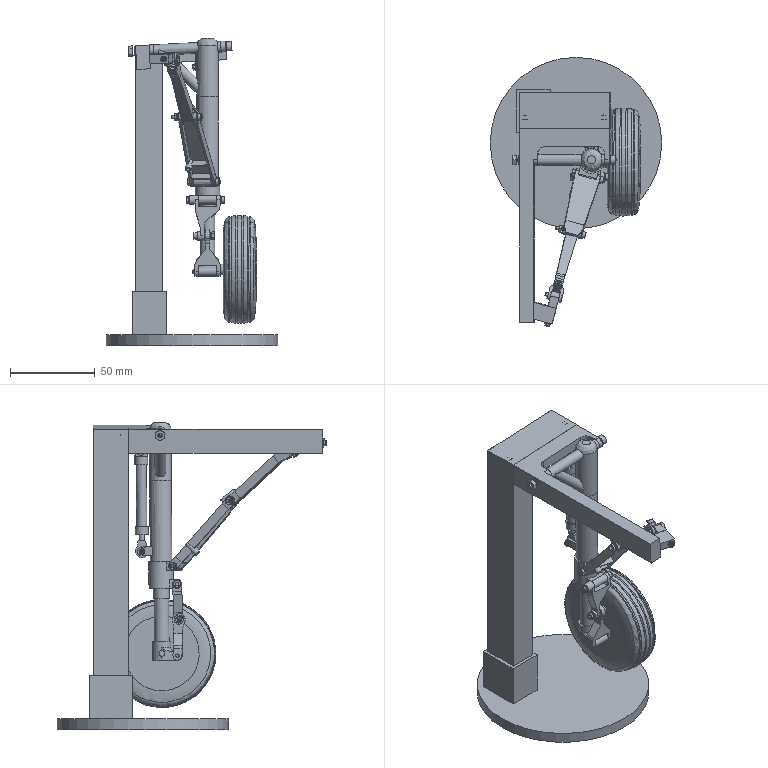Assembly | NX | mm | 58 component files | 58 solids | 973 faces | box 101 x 158.93 x 181.11 mm | volume 209079 mm3 | plane 512 | cone 218 | cylinder 196 | torus 33 | spline 10 | sphere 4 | commonest cylinder face diameters 2 x26 5.292 x14 6.35 x14 12.7 x9 3.3 x9 3.35 x8 2.35 x8 1.587 x6
Bill of materials:
GB93-87,2 | 8 |  | Single Coil Spring Lock Washer, Normal Type, GB 93-87,2
GB-T848-2002,M2 | 6 |  | Thin, flat ring (annular disc) with a single concentric through-hole; looks like a plain flat washer.
unnamed part 1 | 1 |  | Y-shaped or triangular plate bracket. Two widely spaced lugs with holes form a forked top, and the body tapers down to a single lug with a hole at the bottom.
unnamed part 2 | 1 |  | Long, slightly tapered channel or frame arm. Twin parallel side plates are joined by cross webs, and each end has a forked pair of lugs with holes. A small cylindrical boss sticks out from one side.
unnamed part 3 | 1 |  | Inverted-L (gamma-shaped) bar of rectangular cross-section: a long vertical leg with a short horizontal arm at the top. Small holes are visible near the corner and at the arm end.
unnamed part 4 | 1 |  | Wheel with tyre: a rounded toroidal tread with several circumferential grooves around a recessed central hub disc that has a small central bore.
GB-T70.1-2000,M2x20 | 1 |  | Hexagon Socket Head Cap Screw, GB-T 70.1-2000,M2x20
unnamed part 5 | 2 |  | Sphere truncated by two parallel flat faces and pierced by a central through-bore along the axis normal to those faces. It resembles a ball-joint ball or bead.
unnamed part 6 | 1 |  | Thin circular disc base with a hollow square tube standing upright on it, offset from the disc centre.
unnamed part 7 | 1 |  | Long rectangular bar with a hook- or C-shaped end. The end returns into a bracket with holed lugs and a slot, and a small angled block with a hole sits near the opposite end.
unnamed part 8 | 1 |  | Clevis or fork bracket: two parallel lugs with coaxial holes rising from a rounded base. The base has a larger cross hole and a U-shaped slot between the lugs.
unnamed part 9 | 1 |  | Hollow cylindrical tube with a pair of small parallel tabs near one end. The tabs have holes and form a small fork on the tube side.
unnamed part 10 | 1 |  | Tubular frame node: a vertical round post with a domed or ball-shaped top. A horizontal round bar passes through the top, and a diagonal brace runs from the bar to the post. A small bossed hole sits on the dome.
GB-T6170_F-2000,M3x0.5 | 1 |  | Hexagonal nut-like body with a central round bore and chamfered corners on both faces.
GB-T119.1-2000,2x10 | 1 |  | Parallel Pin, GB-T 119.1-2000,2x10
GB-T6170_F-2000,M1.6x0.35 | 2 |  | Hexagonal nut-like body with a central round bore and chamfered corners on both faces.
GB93-87,3 | 2 |  | Single Coil Spring Lock Washer, Normal Type, GB 93-87,3
unnamed part 11 | 1 |  | Cylindrical sleeve with a large axial through-bore and two flat lugs with rounded ends sticking out sideways. The lugs sit at different heights and point in slightly different directions, and each has a small through-hole.
unnamed part 12 | 1 |  | Tee-shaped body: a vertical cylindrical boss with an open, hollow top bore, a flat rounded-end lug with a small through-hole, and a short side boss with a larger through-hole. The side boss axis runs at right angles to the vertical boss. The joins between features are smoothly filleted.
unnamed part 13 | 1 |  | Flat Y-shaped forked lever. One end is a single rounded eye with a larger hole. A narrow stem widens into a two-prong fork at the other end, and each prong ends in a rounded tip with a small hole.
unnamed part 14 | 1 |  | Long, straight, thin-walled round tube with plain square-cut ends.
unnamed part 15 | 1 |  | Rectangular block with one end rounded into a semicircle. One through-hole runs across the rounded end, square to the large side faces. A second hole enters the flat square end face.
GB-T119.1-2000,2x16 | 1 |  | Parallel Pin, GB-T 119.1-2000,2x16
unnamed part 16 | 1 |  | Long, straight, thin-walled round tube with plain square-cut ends.
GB-T70.1-2000,M3x30 | 1 |  | Hexagon Socket Head Cap Screw, GB-T 70.1-2000,M3x30
unnamed part 17 | 1 |  | Slender solid round rod with a flat eyelet lug at one end. The lug has a through-hole whose axis is square to the rod axis.
GB-T6170_F-2000,M2x0.4 | 5 |  | Hexagonal prism with a round central through-hole. The corners are chamfered on both faces, which gives curved arcs on the side flats. It looks like a hex nut.
GB-T70.1-2000,M1.6x10 | 3 |  | Hexagon Socket Head Cap Screw, GB-T 70.1-2000,M1.6x10
unnamed part 18 | 1 |  | Slender cylindrical body with a larger-diameter collar at each end. A flat tab with a small cross-hole sticks out from one end collar.
GB-T70.1-2000,M3x5 | 3 |  | Hexagon Socket Head Cap Screw, GB-T 70.1-2000,M3x5
GB-T70.1-2000,M2x16 | 2 |  | Hexagon Socket Head Cap Screw, GB-T 70.1-2000,M2x16
GB-T70.1-2000,M2x10 | 2 |  | Hexagon Socket Head Cap Screw, GB-T 70.1-2000,M2x10
unnamed part 19 | 1 |  | Long, flat, slightly tapered arm. One end is a two-prong fork with a small hole in each prong tip. The other end has a rounded boss with a hole and a stepped, angled tab.
Mates:
1. fix | base 1 component
2. touch align | support_rod 1 face | base 1 face
3. center | support_rod 1 face | support_rod 1 face | base 1 face | base 1 face
4. center | support_rod 1 face | support_rod 1 face | base 1 face | base 1 face
5. concentric | main_frame 1 edge | support_rod 1 edge
6. concentric | bearing_housing 1 edge | main_frame 1 edge
7. concentric | casing 1 edge | bearing_housing 1 edge
8. parallel | main_frame 1 face | support_rod 1 face
9. concentric | connecting_block 1 edge | casing 1 edge
10. concentric | block 1 edge | main_frame 1 edge
11. center | universal_joint_1 1 face | universal_joint_1 1 face | block 1 face | block 1 face
12. touch align | universal_joint_1 1 face | block 1 face
13. center | connecting_rod_2 1 face | connecting_rod_2 1 face | universal_joint_1 1 face | universal_joint_1 1 face
14. touch align | connecting_rod_2 1 face | universal_joint_1 1 face
15. center | connecting_rod 1 face | connecting_rod 1 face | connecting_rod_2 1 face | connecting_rod_2 1 face
16. touch align | connecting_rod 1 face | connecting_rod_2 1 face
17. touch align | connecting_rod 1 face | connecting_block 1 face
18. center | connecting_rod 1 face | connecting_rod 1 face | connecting_block 1 face | connecting_block 1 face
19. touch align | rotating_rod_2 1 face | connecting_block 1 face
20. center | rotating_rod_2 1 face | rotating_rod_2 1 face | connecting_block 1 face | connecting_block 1 face
21. touch align | tube_2 1 face | casing 1 face
22. touch align | tube_1 1 face | tube_2 1 face
23. distance | tube_2 1 face | connecting_block 1 face
24. touch align | support 1 face | tube_1 1 face
25. fit | ball_1 2 face | rotating_rod 1 face
26. center | rotating_rod 1 face | rotating_rod 1 face | support 1 face | support 1 face
27. touch align | rotating_rod 1 face | support 1 face
28. touch align | ball_1 2 face | rotating_rod_2 1 face
29. touch align | tube_1 1 face | support 1 face
30. touch align | cylinder_block 1 face | main_frame 1 face
31. center | cylinder_block 1 face | cylinder_block 1 face | main_frame 1 face | main_frame 1 face
32. concentric | wheel 1 edge | support 1 edge
33. touch align | telescopic_rod_1 1 face | cylinder_block 1 face
34. fit | ball_1 1 face | telescopic_rod_1 1 face
35. touch align | ball_1 1 face | casing 1 face
36. parallel | telescopic_rod_1 1 face | casing 1 face